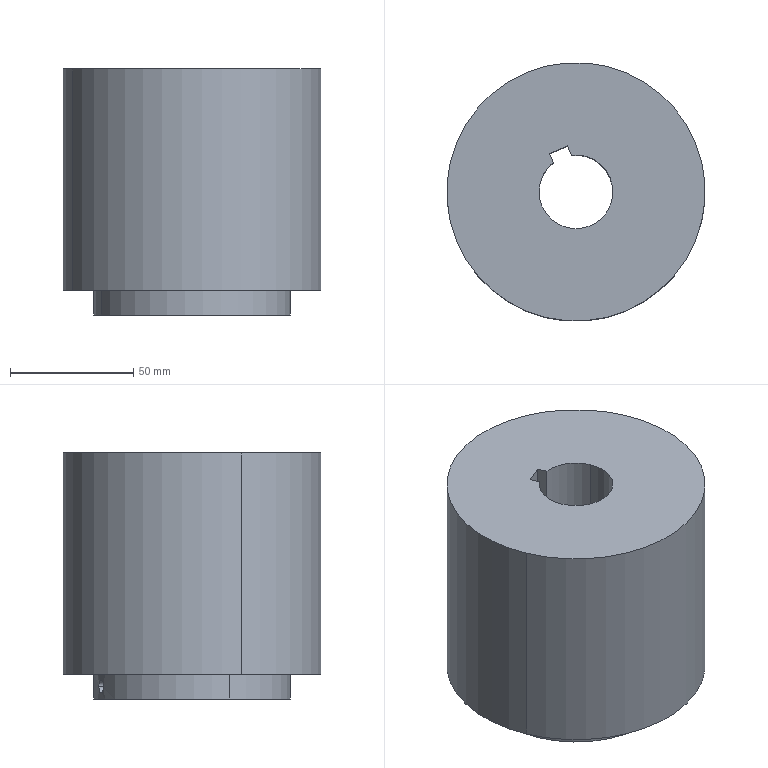Component | SolidWorks | -MainDrivePulley-1 | 1 solid | 15 faces | box 105 x 105 x 100 mm | volume 755525 mm3 | cylinder 9 | plane 6 | commonest cylinder face diameters 30 x3 5 x2 80 x2 105 x2
build123d program:
from build123d import *

# Parameters (mm, degrees)
SKETCH2_W             = 8
SKETCH2_H             = 9.421
CUT_EXTRUDE1_DEPTH    = 125.549
M6_TAPPED_HOLE1_D     = 5
M6_TAPPED_HOLE1_DEPTH = 30
M6_TAPPED_HOLE1_TIP   = 1.502


with BuildPart() as part:
    # Sketch1 → Revolve1 (revolve)
    with BuildSketch(Plane(origin=(0, 0, 0), x_dir=(1, 0, 0), z_dir=(0, 1, 0)), mode=Mode.PRIVATE) as revolve1_sk:
        Polygon((0, 52.5), (90, 52.5), (90, 40), (100, 40), (100, 15), (0, 15), align=None)
    revolve(revolve1_sk.sketch.rotate(Axis((-694.122, 0, 0), (1, 0, 0)), 180), axis=Axis((-694.122, 0, 0), (1, 0, 0)))

    # Sketch2 → Cut-Extrude1 (cut, through all)
    with BuildSketch(Plane(origin=(100, 0, 0), x_dir=(0, 0, -1), z_dir=(1, 0, 0))):
        with Locations((0, 13.789)):
            Rectangle(SKETCH2_W, SKETCH2_H)
    extrude(amount=-CUT_EXTRUDE1_DEPTH, mode=Mode.SUBTRACT)

    # M6 Tapped Hole1
    with Locations(Plane(origin=(0, 40, 0), x_dir=(1, 0, 0), z_dir=(0, 1, 0))):
        with Locations((95, 0)):
            Hole(M6_TAPPED_HOLE1_D / 2, depth=M6_TAPPED_HOLE1_DEPTH)
            with Locations((0, 0, -(M6_TAPPED_HOLE1_DEPTH + M6_TAPPED_HOLE1_TIP / 2))):  # 118° drill point
                Cone(0, M6_TAPPED_HOLE1_D / 2, M6_TAPPED_HOLE1_TIP, mode=Mode.SUBTRACT)


solid = part.part

# Placed as in the assembly
solid = solid.moved(Location((205, 1094.5, 135), (-90.001, 67.481, 90)))
STEP:
#1=CARTESIAN_POINT('',(7.701,43.726,1.575));
#2=VERTEX_POINT('',#1);
#3=CARTESIAN_POINT('',(7.883,43.801,1.575));
#4=VERTEX_POINT('',#3);
#5=CARTESIAN_POINT('',(7.792,43.763,1.575));
#6=DIRECTION('',(-0.383,0.9237,-0.));
#7=DIRECTION('',(0.9237,0.383,0.));
#8=AXIS2_PLACEMENT_3D('',#5,#6,#7);
#9=CIRCLE('',#8,0.09843);
#10=EDGE_CURVE('',#2,#4,#9,.T.);
#11=ORIENTED_EDGE('',*,*,#10,.F.);
#12=CARTESIAN_POINT('',(7.378,44.505,1.575));
#13=VERTEX_POINT('',#12);
#14=CARTESIAN_POINT('',(7.377,44.508,1.575));
#15=DIRECTION('',(-0.383,0.9237,-0.));
#16=VECTOR('',#15,39.37);
#17=LINE('',#14,#16);
#18=EDGE_CURVE('',#2,#13,#17,.T.);
#19=ORIENTED_EDGE('',*,*,#18,.T.);
#20=CARTESIAN_POINT('',(7.56,44.58,1.575));
#21=VERTEX_POINT('',#20);
#22=CARTESIAN_POINT('',(7.56,44.58,1.575));
#23=CARTESIAN_POINT('',(7.56,44.58,1.581));
#24=CARTESIAN_POINT('',(7.559,44.58,1.588));
#25=CARTESIAN_POINT('',(7.557,44.579,1.6));
#26=CARTESIAN_POINT('',(7.555,44.578,1.607));
#27=CARTESIAN_POINT('',(7.55,44.577,1.618));
#28=CARTESIAN_POINT('',(7.547,44.576,1.624));
#29=CARTESIAN_POINT('',(7.541,44.573,1.635));
#30=CARTESIAN_POINT('',(7.537,44.572,1.64));
#31=CARTESIAN_POINT('',(7.528,44.569,1.649));
#32=CARTESIAN_POINT('',(7.524,44.567,1.653));
#33=CARTESIAN_POINT('',(7.513,44.563,1.66));
#34=CARTESIAN_POINT('',(7.508,44.561,1.663));
#35=CARTESIAN_POINT('',(7.497,44.557,1.668));
#36=CARTESIAN_POINT('',(7.491,44.555,1.67));
#37=CARTESIAN_POINT('',(7.48,44.55,1.673));
#38=CARTESIAN_POINT('',(7.474,44.548,1.673));
#39=CARTESIAN_POINT('',(7.462,44.543,1.673));
#40=CARTESIAN_POINT('',(7.456,44.54,1.673));
#41=CARTESIAN_POINT('',(7.444,44.535,1.67));
#42=CARTESIAN_POINT('',(7.439,44.533,1.668));
#43=CARTESIAN_POINT('',(7.428,44.528,1.663));
#44=CARTESIAN_POINT('',(7.422,44.526,1.66));
#45=CARTESIAN_POINT('',(7.413,44.521,1.653));
#46=CARTESIAN_POINT('',(7.408,44.519,1.649));
#47=CARTESIAN_POINT('',(7.4,44.515,1.64));
#48=CARTESIAN_POINT('',(7.396,44.513,1.635));
#49=CARTESIAN_POINT('',(7.39,44.51,1.624));
#50=CARTESIAN_POINT('',(7.387,44.509,1.618));
#51=CARTESIAN_POINT('',(7.382,44.507,1.607));
#52=CARTESIAN_POINT('',(7.381,44.506,1.6));
#53=CARTESIAN_POINT('',(7.378,44.505,1.588));
#54=CARTESIAN_POINT('',(7.378,44.505,1.581));
#55=CARTESIAN_POINT('',(7.378,44.505,1.575));
#56=B_SPLINE_CURVE_WITH_KNOTS('',3,(#22,#23,#24,#25,#26,#27,#28,#29,#30,#31,#32,#33,#34,#35,#36,#37,#38,#39,#40,#41,#42,#43,#44,#45,#46,#47,#48,#49,#50,#51,#52,#53,#54,#55),.UNSPECIFIED.,.F.,.F.,(4,2,2,2,2,2,2,2,2,2,2,2,2,2,2,2,4),(0.,0.0004886,0.0009773,0.001466,0.001955,0.002443,0.002932,0.00342,0.003909,0.004398,0.004886,0.005375,0.005864,0.006352,0.006841,0.007329,0.007818),.UNSPECIFIED.);
#57=EDGE_CURVE('',#21,#13,#56,.T.);
#58=ORIENTED_EDGE('',*,*,#57,.F.);
#59=CARTESIAN_POINT('',(7.559,44.583,1.575));
#60=DIRECTION('',(-0.383,0.9237,-0.));
#61=VECTOR('',#60,39.37);
#62=LINE('',#59,#61);
#63=EDGE_CURVE('',#4,#21,#62,.T.);
#64=ORIENTED_EDGE('',*,*,#63,.F.);
#65=EDGE_LOOP('',(#11,#19,#58,#64));
#66=FACE_OUTER_BOUND('',#65,.T.);
#67=CARTESIAN_POINT('',(7.468,44.545,1.575));
#68=DIRECTION('',(-0.383,0.9237,-0.));
#69=DIRECTION('',(0.9237,0.383,0.));
#70=AXIS2_PLACEMENT_3D('',#67,#68,#69);
#71=CYLINDRICAL_SURFACE('',#70,0.09843);
#72=ADVANCED_FACE('',(#66),#71,.F.);
#73=CARTESIAN_POINT('',(7.525,42.864,1.378));
#74=VERTEX_POINT('',#73);
#75=CARTESIAN_POINT('',(8.616,43.317,1.378));
#76=VERTEX_POINT('',#75);
#77=CARTESIAN_POINT('',(8.071,43.091,1.378));
#78=DIRECTION('',(0.,0.,1.));
#79=DIRECTION('',(0.9237,0.383,-0.));
#80=AXIS2_PLACEMENT_3D('',#77,#78,#79);
#81=CIRCLE('',#80,0.5906);
#82=EDGE_CURVE('',#74,#76,#81,.T.);
#83=ORIENTED_EDGE('',*,*,#82,.F.);
#84=CARTESIAN_POINT('',(7.525,42.864,5.315));
#85=VERTEX_POINT('',#84);
#86=CARTESIAN_POINT('',(7.525,42.864,32.643));
#87=DIRECTION('',(0.,0.,1.));
#88=VECTOR('',#87,39.37);
#89=LINE('',#86,#88);
#90=EDGE_CURVE('',#74,#85,#89,.T.);
#91=ORIENTED_EDGE('',*,*,#90,.T.);
#92=CARTESIAN_POINT('',(8.616,43.317,5.315));
#93=VERTEX_POINT('',#92);
#94=CARTESIAN_POINT('',(8.071,43.091,5.315));
#95=DIRECTION('',(0.,0.,1.));
#96=DIRECTION('',(0.9237,0.383,0.));
#97=AXIS2_PLACEMENT_3D('',#94,#95,#96);
#98=CIRCLE('',#97,0.5906);
#99=EDGE_CURVE('',#85,#93,#98,.T.);
#100=ORIENTED_EDGE('',*,*,#99,.T.);
#101=CARTESIAN_POINT('',(8.616,43.317,32.643));
#102=DIRECTION('',(0.,0.,1.));
#103=VECTOR('',#102,39.37);
#104=LINE('',#101,#103);
#105=EDGE_CURVE('',#76,#93,#104,.T.);
#106=ORIENTED_EDGE('',*,*,#105,.F.);
#107=EDGE_LOOP('',(#83,#91,#100,#106));
#108=FACE_OUTER_BOUND('',#107,.T.);
#109=CARTESIAN_POINT('',(8.071,43.091,32.643));
#110=DIRECTION('',(0.,0.,1.));
#111=DIRECTION('',(0.9237,0.383,0.));
#112=AXIS2_PLACEMENT_3D('',#109,#110,#111);
#113=CYLINDRICAL_SURFACE('',#112,0.5906);
#114=ADVANCED_FACE('',(#108),#113,.F.);
#115=CARTESIAN_POINT('',(7.998,43.677,1.378));
#116=VERTEX_POINT('',#115);
#117=CARTESIAN_POINT('',(8.071,43.091,1.378));
#118=DIRECTION('',(0.,0.,1.));
#119=DIRECTION('',(0.9237,0.383,-0.));
#120=AXIS2_PLACEMENT_3D('',#117,#118,#119);
#121=CIRCLE('',#120,0.5906);
#122=EDGE_CURVE('',#76,#116,#121,.T.);
#123=ORIENTED_EDGE('',*,*,#122,.F.);
#124=ORIENTED_EDGE('',*,*,#105,.T.);
#125=CARTESIAN_POINT('',(7.998,43.677,5.315));
#126=VERTEX_POINT('',#125);
#127=CARTESIAN_POINT('',(8.071,43.091,5.315));
#128=DIRECTION('',(0.,0.,1.));
#129=DIRECTION('',(0.9237,0.383,0.));
#130=AXIS2_PLACEMENT_3D('',#127,#128,#129);
#131=CIRCLE('',#130,0.5906);
#132=EDGE_CURVE('',#93,#126,#131,.T.);
#133=ORIENTED_EDGE('',*,*,#132,.T.);
#134=CARTESIAN_POINT('',(7.998,43.677,32.643));
#135=DIRECTION('',(-0.,-0.,-1.));
#136=VECTOR('',#135,39.37);
#137=LINE('',#134,#136);
#138=EDGE_CURVE('',#126,#116,#137,.T.);
#139=ORIENTED_EDGE('',*,*,#138,.T.);
#140=EDGE_LOOP('',(#123,#124,#133,#139));
#141=FACE_OUTER_BOUND('',#140,.T.);
#142=CARTESIAN_POINT('',(8.071,43.091,32.643));
#143=DIRECTION('',(0.,0.,1.));
#144=DIRECTION('',(0.9237,0.383,0.));
#145=AXIS2_PLACEMENT_3D('',#142,#143,#144);
#146=CYLINDRICAL_SURFACE('',#145,0.5906);
#147=ADVANCED_FACE('',(#141),#146,.F.);
#148=ORIENTED_EDGE('',*,*,#57,.T.);
#149=CARTESIAN_POINT('',(7.378,44.505,1.575));
#150=CARTESIAN_POINT('',(7.378,44.505,1.568));
#151=CARTESIAN_POINT('',(7.378,44.505,1.562));
#152=CARTESIAN_POINT('',(7.381,44.506,1.549));
#153=CARTESIAN_POINT('',(7.382,44.507,1.543));
#154=CARTESIAN_POINT('',(7.389,44.51,1.525));
#155=CARTESIAN_POINT('',(7.396,44.513,1.514));
#156=CARTESIAN_POINT('',(7.408,44.519,1.501));
#157=CARTESIAN_POINT('',(7.413,44.521,1.497));
#158=CARTESIAN_POINT('',(7.422,44.526,1.489));
#159=CARTESIAN_POINT('',(7.427,44.528,1.486));
#160=CARTESIAN_POINT('',(7.438,44.533,1.481));
#161=CARTESIAN_POINT('',(7.444,44.535,1.48));
#162=CARTESIAN_POINT('',(7.456,44.54,1.477));
#163=CARTESIAN_POINT('',(7.462,44.543,1.476));
#164=CARTESIAN_POINT('',(7.474,44.548,1.476));
#165=CARTESIAN_POINT('',(7.48,44.55,1.477));
#166=CARTESIAN_POINT('',(7.491,44.555,1.479));
#167=CARTESIAN_POINT('',(7.497,44.557,1.481));
#168=CARTESIAN_POINT('',(7.508,44.561,1.486));
#169=CARTESIAN_POINT('',(7.513,44.563,1.489));
#170=CARTESIAN_POINT('',(7.523,44.567,1.496));
#171=CARTESIAN_POINT('',(7.528,44.569,1.501));
#172=CARTESIAN_POINT('',(7.537,44.572,1.51));
#173=CARTESIAN_POINT('',(7.541,44.573,1.515));
#174=CARTESIAN_POINT('',(7.547,44.576,1.525));
#175=CARTESIAN_POINT('',(7.55,44.577,1.531));
#176=CARTESIAN_POINT('',(7.557,44.579,1.549));
#177=CARTESIAN_POINT('',(7.56,44.58,1.562));
#178=CARTESIAN_POINT('',(7.56,44.58,1.575));
#179=B_SPLINE_CURVE_WITH_KNOTS('',3,(#149,#150,#151,#152,#153,#154,#155,#156,#157,#158,#159,#160,#161,#162,#163,#164,#165,#166,#167,#168,#169,#170,#171,#172,#173,#174,#175,#176,#177,#178),.UNSPECIFIED.,.F.,.F.,(4,2,2,2,2,2,2,2,2,2,2,2,2,2,4),(0.007818,0.008307,0.008795,0.009772,0.01026,0.01075,0.01124,0.01173,0.01221,0.0127,0.01319,0.01368,0.01417,0.01466,0.01563),.UNSPECIFIED.);
#180=EDGE_CURVE('',#13,#21,#179,.T.);
#181=ORIENTED_EDGE('',*,*,#180,.T.);
#182=EDGE_LOOP('',(#148,#181));
#183=FACE_BOUND('',#182,.T.);
#184=CARTESIAN_POINT('',(9.526,43.694,1.378));
#185=VERTEX_POINT('',#184);
#186=CARTESIAN_POINT('',(6.616,42.487,1.378));
#187=VERTEX_POINT('',#186);
#188=CARTESIAN_POINT('',(8.071,43.091,1.378));
#189=DIRECTION('',(0.,0.,1.));
#190=DIRECTION('',(0.9237,0.383,-0.));
#191=AXIS2_PLACEMENT_3D('',#188,#189,#190);
#192=CIRCLE('',#191,1.575);
#193=EDGE_CURVE('',#185,#187,#192,.T.);
#194=ORIENTED_EDGE('',*,*,#193,.T.);
#195=CARTESIAN_POINT('',(6.616,42.487,1.772));
#196=VERTEX_POINT('',#195);
#197=CARTESIAN_POINT('',(6.616,42.487,32.643));
#198=DIRECTION('',(0.,0.,1.));
#199=VECTOR('',#198,39.37);
#200=LINE('',#197,#199);
#201=EDGE_CURVE('',#187,#196,#200,.T.);
#202=ORIENTED_EDGE('',*,*,#201,.T.);
#203=CARTESIAN_POINT('',(9.526,43.694,1.772));
#204=VERTEX_POINT('',#203);
#205=CARTESIAN_POINT('',(8.071,43.091,1.772));
#206=DIRECTION('',(0.,0.,1.));
#207=DIRECTION('',(0.9237,0.383,-0.));
#208=AXIS2_PLACEMENT_3D('',#205,#206,#207);
#209=CIRCLE('',#208,1.575);
#210=EDGE_CURVE('',#204,#196,#209,.T.);
#211=ORIENTED_EDGE('',*,*,#210,.F.);
#212=CARTESIAN_POINT('',(9.526,43.694,32.643));
#213=DIRECTION('',(0.,0.,1.));
#214=VECTOR('',#213,39.37);
#215=LINE('',#212,#214);
#216=EDGE_CURVE('',#185,#204,#215,.T.);
#217=ORIENTED_EDGE('',*,*,#216,.F.);
#218=EDGE_LOOP('',(#194,#202,#211,#217));
#219=FACE_OUTER_BOUND('',#218,.T.);
#220=CARTESIAN_POINT('',(8.071,43.091,32.643));
#221=DIRECTION('',(0.,0.,1.));
#222=DIRECTION('',(0.9237,0.383,0.));
#223=AXIS2_PLACEMENT_3D('',#220,#221,#222);
#224=CYLINDRICAL_SURFACE('',#223,1.575);
#225=ADVANCED_FACE('',(#183,#219),#224,.T.);
#226=CARTESIAN_POINT('',(9.98,43.882,1.772));
#227=VERTEX_POINT('',#226);
#228=CARTESIAN_POINT('',(6.162,42.299,1.772));
#229=VERTEX_POINT('',#228);
#230=CARTESIAN_POINT('',(8.071,43.091,1.772));
#231=DIRECTION('',(0.,0.,1.));
#232=DIRECTION('',(0.9237,0.383,-0.));
#233=AXIS2_PLACEMENT_3D('',#230,#231,#232);
#234=CIRCLE('',#233,2.067);
#235=EDGE_CURVE('',#227,#229,#234,.T.);
#236=ORIENTED_EDGE('',*,*,#235,.T.);
#237=CARTESIAN_POINT('',(6.162,42.299,5.315));
#238=VERTEX_POINT('',#237);
#239=CARTESIAN_POINT('',(6.162,42.299,32.643));
#240=DIRECTION('',(0.,0.,1.));
#241=VECTOR('',#240,39.37);
#242=LINE('',#239,#241);
#243=EDGE_CURVE('',#229,#238,#242,.T.);
#244=ORIENTED_EDGE('',*,*,#243,.T.);
#245=CARTESIAN_POINT('',(9.98,43.882,5.315));
#246=VERTEX_POINT('',#245);
#247=CARTESIAN_POINT('',(8.071,43.091,5.315));
#248=DIRECTION('',(0.,0.,1.));
#249=DIRECTION('',(0.9237,0.383,-0.));
#250=AXIS2_PLACEMENT_3D('',#247,#248,#249);
#251=CIRCLE('',#250,2.067);
#252=EDGE_CURVE('',#246,#238,#251,.T.);
#253=ORIENTED_EDGE('',*,*,#252,.F.);
#254=CARTESIAN_POINT('',(9.98,43.882,32.643));
#255=DIRECTION('',(0.,0.,1.));
#256=VECTOR('',#255,39.37);
#257=LINE('',#254,#256);
#258=EDGE_CURVE('',#227,#246,#257,.T.);
#259=ORIENTED_EDGE('',*,*,#258,.F.);
#260=EDGE_LOOP('',(#236,#244,#253,#259));
#261=FACE_OUTER_BOUND('',#260,.T.);
#262=CARTESIAN_POINT('',(8.071,43.091,32.643));
#263=DIRECTION('',(0.,0.,1.));
#264=DIRECTION('',(0.9237,0.383,0.));
#265=AXIS2_PLACEMENT_3D('',#262,#263,#264);
#266=CYLINDRICAL_SURFACE('',#265,2.067);
#267=ADVANCED_FACE('',(#261),#266,.T.);
#268=CARTESIAN_POINT('',(7.646,43.703,5.315));
#269=VERTEX_POINT('',#268);
#270=CARTESIAN_POINT('',(7.937,43.824,5.315));
#271=VERTEX_POINT('',#270);
#272=CARTESIAN_POINT('',(7.937,43.824,5.315));
#273=DIRECTION('',(0.9237,0.383,-0.));
#274=VECTOR('',#273,39.37);
#275=LINE('',#272,#274);
#276=EDGE_CURVE('',#269,#271,#275,.T.);
#277=ORIENTED_EDGE('',*,*,#276,.T.);
#278=CARTESIAN_POINT('',(7.937,43.824,5.315));
#279=DIRECTION('',(0.383,-0.9237,0.));
#280=VECTOR('',#279,39.37);
#281=LINE('',#278,#280);
#282=EDGE_CURVE('',#271,#126,#281,.T.);
#283=ORIENTED_EDGE('',*,*,#282,.T.);
#284=ORIENTED_EDGE('',*,*,#132,.F.);
#285=ORIENTED_EDGE('',*,*,#99,.F.);
#286=CARTESIAN_POINT('',(7.707,43.556,5.315));
#287=VERTEX_POINT('',#286);
#288=CARTESIAN_POINT('',(8.071,43.091,5.315));
#289=DIRECTION('',(0.,0.,1.));
#290=DIRECTION('',(0.9237,0.383,0.));
#291=AXIS2_PLACEMENT_3D('',#288,#289,#290);
#292=CIRCLE('',#291,0.5906);
#293=EDGE_CURVE('',#287,#85,#292,.T.);
#294=ORIENTED_EDGE('',*,*,#293,.F.);
#295=CARTESIAN_POINT('',(7.646,43.703,5.315));
#296=DIRECTION('',(-0.383,0.9237,-0.));
#297=VECTOR('',#296,39.37);
#298=LINE('',#295,#297);
#299=EDGE_CURVE('',#287,#269,#298,.T.);
#300=ORIENTED_EDGE('',*,*,#299,.T.);
#301=EDGE_LOOP('',(#277,#283,#284,#285,#294,#300));
#302=FACE_BOUND('',#301,.T.);
#303=ORIENTED_EDGE('',*,*,#252,.T.);
#304=CARTESIAN_POINT('',(8.071,43.091,5.315));
#305=DIRECTION('',(0.,0.,1.));
#306=DIRECTION('',(0.9237,0.383,-0.));
#307=AXIS2_PLACEMENT_3D('',#304,#305,#306);
#308=CIRCLE('',#307,2.067);
#309=EDGE_CURVE('',#238,#246,#308,.T.);
#310=ORIENTED_EDGE('',*,*,#309,.T.);
#311=EDGE_LOOP('',(#303,#310));
#312=FACE_OUTER_BOUND('',#311,.T.);
#313=CARTESIAN_POINT('',(7.525,42.864,5.315));
#314=DIRECTION('',(-0.,-0.,-1.));
#315=DIRECTION('',(-0.9237,-0.383,0.));
#316=AXIS2_PLACEMENT_3D('',#313,#314,#315);
#317=PLANE('',#316);
#318=ADVANCED_FACE('',(#302,#312),#317,.F.);
#319=ORIENTED_EDGE('',*,*,#243,.F.);
#320=CARTESIAN_POINT('',(8.071,43.091,1.772));
#321=DIRECTION('',(0.,0.,1.));
#322=DIRECTION('',(0.9237,0.383,-0.));
#323=AXIS2_PLACEMENT_3D('',#320,#321,#322);
#324=CIRCLE('',#323,2.067);
#325=EDGE_CURVE('',#229,#227,#324,.T.);
#326=ORIENTED_EDGE('',*,*,#325,.T.);
#327=ORIENTED_EDGE('',*,*,#258,.T.);
#328=ORIENTED_EDGE('',*,*,#309,.F.);
#329=EDGE_LOOP('',(#319,#326,#327,#328));
#330=FACE_OUTER_BOUND('',#329,.T.);
#331=CARTESIAN_POINT('',(8.071,43.091,32.643));
#332=DIRECTION('',(0.,0.,1.));
#333=DIRECTION('',(0.9237,0.383,0.));
#334=AXIS2_PLACEMENT_3D('',#331,#332,#333);
#335=CYLINDRICAL_SURFACE('',#334,2.067);
#336=ADVANCED_FACE('',(#330),#335,.T.);
#337=ORIENTED_EDGE('',*,*,#235,.F.);
#338=ORIENTED_EDGE('',*,*,#325,.F.);
#339=EDGE_LOOP('',(#337,#338));
#340=FACE_OUTER_BOUND('',#339,.T.);
#341=ORIENTED_EDGE('',*,*,#210,.T.);
#342=CARTESIAN_POINT('',(8.071,43.091,1.772));
#343=DIRECTION('',(0.,0.,1.));
#344=DIRECTION('',(0.9237,0.383,-0.));
#345=AXIS2_PLACEMENT_3D('',#342,#343,#344);
#346=CIRCLE('',#345,1.575);
#347=EDGE_CURVE('',#196,#204,#346,.T.);
#348=ORIENTED_EDGE('',*,*,#347,.T.);
#349=EDGE_LOOP('',(#341,#348));
#350=FACE_BOUND('',#349,.T.);
#351=CARTESIAN_POINT('',(6.162,42.299,1.772));
#352=DIRECTION('',(0.,0.,1.));
#353=DIRECTION('',(0.9237,0.383,-0.));
#354=AXIS2_PLACEMENT_3D('',#351,#352,#353);
#355=PLANE('',#354);
#356=ADVANCED_FACE('',(#340,#350),#355,.F.);
#357=ORIENTED_EDGE('',*,*,#201,.F.);
#358=CARTESIAN_POINT('',(8.071,43.091,1.378));
#359=DIRECTION('',(0.,0.,1.));
#360=DIRECTION('',(0.9237,0.383,-0.));
#361=AXIS2_PLACEMENT_3D('',#358,#359,#360);
#362=CIRCLE('',#361,1.575);
#363=EDGE_CURVE('',#187,#185,#362,.T.);
#364=ORIENTED_EDGE('',*,*,#363,.T.);
#365=ORIENTED_EDGE('',*,*,#216,.T.);
#366=ORIENTED_EDGE('',*,*,#347,.F.);
#367=EDGE_LOOP('',(#357,#364,#365,#366));
#368=FACE_OUTER_BOUND('',#367,.T.);
#369=CARTESIAN_POINT('',(8.071,43.091,32.643));
#370=DIRECTION('',(0.,0.,1.));
#371=DIRECTION('',(0.9237,0.383,0.));
#372=AXIS2_PLACEMENT_3D('',#369,#370,#371);
#373=CYLINDRICAL_SURFACE('',#372,1.575);
#374=ADVANCED_FACE('',(#368),#373,.T.);
#375=ORIENTED_EDGE('',*,*,#193,.F.);
#376=ORIENTED_EDGE('',*,*,#363,.F.);
#377=EDGE_LOOP('',(#375,#376));
#378=FACE_OUTER_BOUND('',#377,.T.);
#379=CARTESIAN_POINT('',(7.707,43.556,1.378));
#380=VERTEX_POINT('',#379);
#381=CARTESIAN_POINT('',(8.071,43.091,1.378));
#382=DIRECTION('',(0.,0.,1.));
#383=DIRECTION('',(0.9237,0.383,-0.));
#384=AXIS2_PLACEMENT_3D('',#381,#382,#383);
#385=CIRCLE('',#384,0.5906);
#386=EDGE_CURVE('',#380,#74,#385,.T.);
#387=ORIENTED_EDGE('',*,*,#386,.T.);
#388=ORIENTED_EDGE('',*,*,#82,.T.);
#389=ORIENTED_EDGE('',*,*,#122,.T.);
#390=CARTESIAN_POINT('',(7.937,43.824,1.378));
#391=VERTEX_POINT('',#390);
#392=CARTESIAN_POINT('',(7.937,43.824,1.378));
#393=DIRECTION('',(0.383,-0.9237,0.));
#394=VECTOR('',#393,39.37);
#395=LINE('',#392,#394);
#396=EDGE_CURVE('',#391,#116,#395,.T.);
#397=ORIENTED_EDGE('',*,*,#396,.F.);
#398=CARTESIAN_POINT('',(7.646,43.703,1.378));
#399=VERTEX_POINT('',#398);
#400=CARTESIAN_POINT('',(7.937,43.824,1.378));
#401=DIRECTION('',(0.9237,0.383,-0.));
#402=VECTOR('',#401,39.37);
#403=LINE('',#400,#402);
#404=EDGE_CURVE('',#399,#391,#403,.T.);
#405=ORIENTED_EDGE('',*,*,#404,.F.);
#406=CARTESIAN_POINT('',(7.646,43.703,1.378));
#407=DIRECTION('',(-0.383,0.9237,-0.));
#408=VECTOR('',#407,39.37);
#409=LINE('',#406,#408);
#410=EDGE_CURVE('',#380,#399,#409,.T.);
#411=ORIENTED_EDGE('',*,*,#410,.F.);
#412=EDGE_LOOP('',(#387,#388,#389,#397,#405,#411));
#413=FACE_BOUND('',#412,.T.);
#414=CARTESIAN_POINT('',(6.616,42.487,1.378));
#415=DIRECTION('',(0.,0.,1.));
#416=DIRECTION('',(0.9237,0.383,-0.));
#417=AXIS2_PLACEMENT_3D('',#414,#415,#416);
#418=PLANE('',#417);
#419=ADVANCED_FACE('',(#378,#413),#418,.F.);
#420=ORIENTED_EDGE('',*,*,#90,.F.);
#421=ORIENTED_EDGE('',*,*,#386,.F.);
#422=CARTESIAN_POINT('',(7.707,43.556,32.643));
#423=DIRECTION('',(0.,0.,1.));
#424=VECTOR('',#423,39.37);
#425=LINE('',#422,#424);
#426=EDGE_CURVE('',#380,#287,#425,.T.);
#427=ORIENTED_EDGE('',*,*,#426,.T.);
#428=ORIENTED_EDGE('',*,*,#293,.T.);
#429=EDGE_LOOP('',(#420,#421,#427,#428));
#430=FACE_OUTER_BOUND('',#429,.T.);
#431=CARTESIAN_POINT('',(8.071,43.091,32.643));
#432=DIRECTION('',(0.,0.,1.));
#433=DIRECTION('',(0.9237,0.383,0.));
#434=AXIS2_PLACEMENT_3D('',#431,#432,#433);
#435=CYLINDRICAL_SURFACE('',#434,0.5906);
#436=ADVANCED_FACE('',(#430),#435,.F.);
#437=ORIENTED_EDGE('',*,*,#282,.F.);
#438=CARTESIAN_POINT('',(7.937,43.824,5.315));
#439=DIRECTION('',(-0.,-0.,-1.));
#440=VECTOR('',#439,39.37);
#441=LINE('',#438,#440);
#442=EDGE_CURVE('',#271,#391,#441,.T.);
#443=ORIENTED_EDGE('',*,*,#442,.T.);
#444=ORIENTED_EDGE('',*,*,#396,.T.);
#445=ORIENTED_EDGE('',*,*,#138,.F.);
#446=EDGE_LOOP('',(#437,#443,#444,#445));
#447=FACE_OUTER_BOUND('',#446,.T.);
#448=CARTESIAN_POINT('',(7.937,43.824,5.315));
#449=DIRECTION('',(0.9237,0.383,-0.));
#450=DIRECTION('',(0.383,-0.9237,0.));
#451=AXIS2_PLACEMENT_3D('',#448,#449,#450);
#452=PLANE('',#451);
#453=ADVANCED_FACE('',(#447),#452,.F.);
#454=ORIENTED_EDGE('',*,*,#410,.T.);
#455=CARTESIAN_POINT('',(7.646,43.703,5.315));
#456=DIRECTION('',(-0.,-0.,-1.));
#457=VECTOR('',#456,39.37);
#458=LINE('',#455,#457);
#459=EDGE_CURVE('',#269,#399,#458,.T.);
#460=ORIENTED_EDGE('',*,*,#459,.F.);
#461=ORIENTED_EDGE('',*,*,#299,.F.);
#462=ORIENTED_EDGE('',*,*,#426,.F.);
#463=EDGE_LOOP('',(#454,#460,#461,#462));
#464=FACE_OUTER_BOUND('',#463,.T.);
#465=CARTESIAN_POINT('',(7.646,43.703,5.315));
#466=DIRECTION('',(-0.9237,-0.383,0.));
#467=DIRECTION('',(-0.383,0.9237,-0.));
#468=AXIS2_PLACEMENT_3D('',#465,#466,#467);
#469=PLANE('',#468);
#470=ADVANCED_FACE('',(#464),#469,.F.);
#471=CARTESIAN_POINT('',(7.792,43.763,1.575));
#472=DIRECTION('',(-0.383,0.9237,-0.));
#473=DIRECTION('',(0.9237,0.383,0.));
#474=AXIS2_PLACEMENT_3D('',#471,#472,#473);
#475=CIRCLE('',#474,0.09843);
#476=EDGE_CURVE('',#4,#2,#475,.T.);
#477=ORIENTED_EDGE('',*,*,#476,.T.);
#478=ORIENTED_EDGE('',*,*,#10,.T.);
#479=EDGE_LOOP('',(#477,#478));
#480=FACE_BOUND('',#479,.T.);
#481=ORIENTED_EDGE('',*,*,#404,.T.);
#482=ORIENTED_EDGE('',*,*,#442,.F.);
#483=ORIENTED_EDGE('',*,*,#276,.F.);
#484=ORIENTED_EDGE('',*,*,#459,.T.);
#485=EDGE_LOOP('',(#481,#482,#483,#484));
#486=FACE_OUTER_BOUND('',#485,.T.);
#487=CARTESIAN_POINT('',(7.937,43.824,5.315));
#488=DIRECTION('',(-0.383,0.9237,-0.));
#489=DIRECTION('',(0.9237,0.383,-0.));
#490=AXIS2_PLACEMENT_3D('',#487,#488,#489);
#491=PLANE('',#490);
#492=ADVANCED_FACE('',(#480,#486),#491,.F.);
#493=ORIENTED_EDGE('',*,*,#18,.F.);
#494=ORIENTED_EDGE('',*,*,#476,.F.);
#495=ORIENTED_EDGE('',*,*,#63,.T.);
#496=ORIENTED_EDGE('',*,*,#180,.F.);
#497=EDGE_LOOP('',(#493,#494,#495,#496));
#498=FACE_OUTER_BOUND('',#497,.T.);
#499=CARTESIAN_POINT('',(7.468,44.545,1.575));
#500=DIRECTION('',(-0.383,0.9237,-0.));
#501=DIRECTION('',(0.9237,0.383,0.));
#502=AXIS2_PLACEMENT_3D('',#499,#500,#501);
#503=CYLINDRICAL_SURFACE('',#502,0.09843);
#504=ADVANCED_FACE('',(#498),#503,.F.);
#505=CLOSED_SHELL('',(#72,#114,#147,#225,#267,#318,#336,#356,#374,#419,#436,#453,#470,#492,#504));
#506=MANIFOLD_SOLID_BREP('',#505);
#507=CARTESIAN_POINT('',(0.,0.,0.));
#508=DIRECTION('',(0.,0.,1.));
#509=DIRECTION('',(1.,0.,0.));
#510=AXIS2_PLACEMENT_3D('',#507,#508,#509);
#511=(LENGTH_UNIT()NAMED_UNIT(*)SI_UNIT($,.METRE.));
#512=LENGTH_MEASURE_WITH_UNIT(LENGTH_MEASURE(0.0254),#511);
#513=DIMENSIONAL_EXPONENTS(1.,0.,0.,0.,0.,0.,0.);
#514=(CONVERSION_BASED_UNIT('',#512)LENGTH_UNIT()NAMED_UNIT(#513));
#515=UNCERTAINTY_MEASURE_WITH_UNIT(LENGTH_MEASURE(0.00001),#514,'','');
#516=(NAMED_UNIT(*)PLANE_ANGLE_UNIT()SI_UNIT($,.RADIAN.));
#517=(NAMED_UNIT(*)SI_UNIT($,.STERADIAN.)SOLID_ANGLE_UNIT());
#518=(GEOMETRIC_REPRESENTATION_CONTEXT(3)GLOBAL_UNCERTAINTY_ASSIGNED_CONTEXT((#515))GLOBAL_UNIT_ASSIGNED_CONTEXT((#514,#516,#517))REPRESENTATION_CONTEXT('',''));
#519=ADVANCED_BREP_SHAPE_REPRESENTATION('',(#506,#510),#518);
#520=COLOUR_RGB('',0.7922,0.8196,0.9333);
#521=FILL_AREA_STYLE_COLOUR('',#520);
#522=FILL_AREA_STYLE('',(#521));
#523=SURFACE_STYLE_FILL_AREA(#522);
#524=SURFACE_SIDE_STYLE('',(#523));
#525=SURFACE_STYLE_USAGE(.BOTH.,#524);
#526=PRESENTATION_STYLE_ASSIGNMENT((#525));
#527=STYLED_ITEM('',(#526),#506);
#528=(LENGTH_UNIT()NAMED_UNIT(*)SI_UNIT($,.METRE.));
#529=LENGTH_MEASURE_WITH_UNIT(LENGTH_MEASURE(0.0254),#528);
#530=DIMENSIONAL_EXPONENTS(1.,0.,0.,0.,0.,0.,0.);
#531=(CONVERSION_BASED_UNIT('',#529)LENGTH_UNIT()NAMED_UNIT(#530));
#532=UNCERTAINTY_MEASURE_WITH_UNIT(LENGTH_MEASURE(0.00001),#531,'','');
#533=(NAMED_UNIT(*)PLANE_ANGLE_UNIT()SI_UNIT($,.RADIAN.));
#534=(NAMED_UNIT(*)SI_UNIT($,.STERADIAN.)SOLID_ANGLE_UNIT());
#535=(GEOMETRIC_REPRESENTATION_CONTEXT(3)GLOBAL_UNCERTAINTY_ASSIGNED_CONTEXT((#532))GLOBAL_UNIT_ASSIGNED_CONTEXT((#531,#533,#534))REPRESENTATION_CONTEXT('',''));
#536=MECHANICAL_DESIGN_GEOMETRIC_PRESENTATION_REPRESENTATION('',(#527),#535);
#537=PRESENTATION_LAYER_ASSIGNMENT('','',(#527));